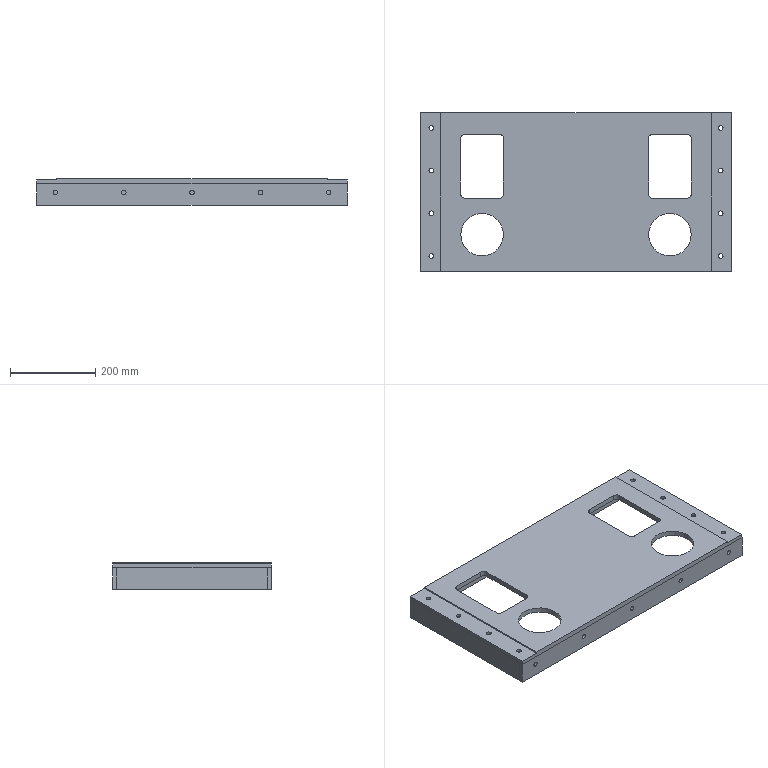Component | SolidWorks | MovingVerticalPlate2-1 | 6 solids | 125 faces | box 728 x 372 x 63 mm | volume 3861761 mm3 | cylinder 64 | plane 61 | commonest cylinder face diameters 18 x26 11 x26 20 x8 100 x4
build123d program:
from build123d import *

# Parameters (mm, degrees)
SKETCH1_W                                  = 728
SKETCH1_H                                  = 372
BOSS_EXTRUDE1_DEPTH                        = 12
SKETCH2_W                                  = 728
SKETCH2_H                                  = 10
BOSS_EXTRUDE2_DEPTH                        = 51
SKETCH3_W                                  = 10
SKETCH3_H                                  = 352
BOSS_EXTRUDE3_DEPTH                        = 51
SKETCH4_W                                  = 10
SKETCH4_H                                  = 352
BOSS_EXTRUDE4_DEPTH                        = 51
HOLE_SIZE_ACCORDING_TO_TYPE_1_OF_H_2_COUNT = 2
HOLE_SIZE_ACCORDING_TO_TYPE_1_OF_H_2_PITCH = 159.546
HOLE_SIZE_ACCORDING_TO_TYPE_1_OF_H_3_COUNT = 2
HOLE_SIZE_ACCORDING_TO_TYPE_1_OF_H_3_PITCH = 320
HOLE_SIZE_ACCORDING_TO_TYPE_1_OF_H_4_COUNT = 2
HOLE_SIZE_ACCORDING_TO_TYPE_1_OF_H_4_PITCH = 480
HOLE_SIZE_ACCORDING_TO_TYPE_1_OF_H_5_COUNT = 2
HOLE_SIZE_ACCORDING_TO_TYPE_1_OF_H_5_PITCH = 640
HOLE_SIZE_ACCORDING_TO_TYPE_2_OF_H_2_COUNT = 2
HOLE_SIZE_ACCORDING_TO_TYPE_2_OF_H_2_PITCH = 100
HOLE_SIZE_ACCORDING_TO_TYPE_2_OF_H_3_COUNT = 2
HOLE_SIZE_ACCORDING_TO_TYPE_2_OF_H_3_PITCH = 200
HOLE_SIZE_ACCORDING_TO_TYPE_2_OF_H_4_COUNT = 2
HOLE_SIZE_ACCORDING_TO_TYPE_2_OF_H_4_PITCH = 300
SKETCH9_R                                  = 50
SKETCH9_W                                  = 100
SKETCH9_H                                  = 150
CUT_EXTRUDE1_DEPTH                         = 412.938
FILLET1_R                                  = 10
SKETCH10_W                                 = 47
SKETCH10_H                                 = 3
CUT_EXTRUDE2_DEPTH                         = 525.26


with BuildPart() as part:
    # Sketch1 → Boss-Extrude1 (new body)
    with BuildSketch(Plane.XY):
        Rectangle(SKETCH1_W, SKETCH1_H)
    extrude(amount=BOSS_EXTRUDE1_DEPTH)

    # Sketch8 → Hole Size _According to_ Type 2 of Hexag (revolve, cut)
    with BuildSketch(Plane(origin=(-339, -150, 12), x_dir=(0, -1, 0), z_dir=(1, 0, 0))):
        Polygon((0, 0), (0, 12), (5.5, 12), (5.5, 3), (9, 3), (9, 0), align=None)
    hole_size_according_to_type_2_of_hexag = revolve(axis=Axis((-339, -150, 18.35), (0, 0, -1)), mode=Mode.SUBTRACT)

    # Hole Size _According to_ Type 2 of H 2: Hole Size _According to_ Type 2 of Hexag ×2
    with Locations(*[(0, i * HOLE_SIZE_ACCORDING_TO_TYPE_2_OF_H_2_PITCH, 0) for i in range(1, HOLE_SIZE_ACCORDING_TO_TYPE_2_OF_H_2_COUNT)]):
        add(hole_size_according_to_type_2_of_hexag, mode=Mode.SUBTRACT)

    # Hole Size _According to_ Type 2 of H 3: Hole Size _According to_ Type 2 of Hexag ×2
    with Locations(*[(0, i * HOLE_SIZE_ACCORDING_TO_TYPE_2_OF_H_3_PITCH, 0) for i in range(1, HOLE_SIZE_ACCORDING_TO_TYPE_2_OF_H_3_COUNT)]):
        add(hole_size_according_to_type_2_of_hexag, mode=Mode.SUBTRACT)

    # Hole Size _According to_ Type 2 of H 4: Hole Size _According to_ Type 2 of Hexag ×2
    with Locations(*[(0, i * HOLE_SIZE_ACCORDING_TO_TYPE_2_OF_H_4_PITCH, 0) for i in range(1, HOLE_SIZE_ACCORDING_TO_TYPE_2_OF_H_4_COUNT)]):
        add(hole_size_according_to_type_2_of_hexag, mode=Mode.SUBTRACT)

    # Mirror3: Hole Size _According to_ Type 2 of Hexag across plane
    add(hole_size_according_to_type_2_of_hexag.mirror(Plane(origin=(0, 0, 0), x_dir=(0, 0, 1), z_dir=(1, 0, 0))), mode=Mode.SUBTRACT)

    # Mirror3 copy 1 sketch → Mirror3 copy 1 (revolve, cut)
    with BuildSketch(Plane(origin=(339, -50, 12), x_dir=(0, -1, 0), z_dir=(-1, 0, 0))):
        Polygon((0, 0), (0, -12), (5.5, -12), (5.5, -3), (9, -3), (9, 0), align=None)
    revolve(axis=Axis((339, -50, 18.35), (0, 0, 1)), mode=Mode.SUBTRACT)

    # Mirror3 copy 2 sketch → Mirror3 copy 2 (revolve, cut)
    with BuildSketch(Plane(origin=(339, 50, 12), x_dir=(0, -1, 0), z_dir=(-1, 0, 0))):
        Polygon((0, 0), (0, -12), (5.5, -12), (5.5, -3), (9, -3), (9, 0), align=None)
    revolve(axis=Axis((339, 50, 18.35), (0, 0, 1)), mode=Mode.SUBTRACT)

    # Mirror3 copy 3 sketch → Mirror3 copy 3 (revolve, cut)
    with BuildSketch(Plane(origin=(339, 150, 12), x_dir=(0, -1, 0), z_dir=(-1, 0, 0))):
        Polygon((0, 0), (0, -12), (5.5, -12), (5.5, -3), (9, -3), (9, 0), align=None)
    revolve(axis=Axis((339, 150, 18.35), (0, 0, 1)), mode=Mode.SUBTRACT)

    # Sketch9 → Cut-Extrude1 (cut, through all)
    with BuildSketch(Plane.XY.offset(12)):
        with Locations((-220, -100)):
            Circle(SKETCH9_R)
        with Locations(Location((220, -100, 0), (0, 0, 180))):
            Circle(SKETCH9_R)
        with Locations((-220, 60)):
            Rectangle(SKETCH9_W, SKETCH9_H)
        with Locations((220, 60)):
            Rectangle(SKETCH9_W, SKETCH9_H)
    extrude(amount=-CUT_EXTRUDE1_DEPTH, mode=Mode.SUBTRACT)

    # Fillet1
    fillet1_edges = [part.edges().sort_by_distance(p)[0] for p in [
        (-270, -15, 6),
        (-270, 135, 6),
        (-170, 135, 6),
        (-170, -15, 6),
        (170, 135, 6),
        (270, 135, 6),
        (270, -15, 6),
        (170, -15, 6),
    ]]
    fillet(fillet1_edges, radius=FILLET1_R)

    # Sketch10 → Cut-Extrude2 (cut, through all)
    with BuildSketch(Plane(origin=(0, 186, 0), x_dir=(1, 0, 0), z_dir=(0, 1, 0))):
        with Locations((340.5, -1.5)):
            Rectangle(SKETCH10_W, SKETCH10_H)
        with Locations((-340.5, -1.5)):
            Rectangle(SKETCH10_W, SKETCH10_H)
    extrude(amount=-CUT_EXTRUDE2_DEPTH, mode=Mode.SUBTRACT)


with BuildPart() as body_2:
    # Sketch2 → Boss-Extrude2 (new body)
    with BuildSketch(Plane.XY.offset(12)):
        with Locations((0, 181)):
            Rectangle(SKETCH2_W, SKETCH2_H)
    extrude(amount=BOSS_EXTRUDE2_DEPTH)


with BuildPart() as body_3:
    # Sketch3 → Boss-Extrude3 (new body)
    with BuildSketch(Plane.XY.offset(12)):
        with Locations((-359, 0)):
            Rectangle(SKETCH3_W, SKETCH3_H)
    extrude(amount=BOSS_EXTRUDE3_DEPTH)


with BuildPart() as body_4:
    # Mirror1: mirrored copy
    add(body_2.part.mirror(Plane.ZX))

    # Sketch6 → Hole Size _According to_ Type 1 of Hexag (revolve, cut)
    with BuildSketch(Plane(origin=(-320, -176, 33), x_dir=(0, 0, 1), z_dir=(1, 0, 0))):
        Polygon((0, 0), (0, 10), (5.5, 10), (5.5, 3), (9, 3), (9, 0), align=None)
    hole_size_according_to_type_1_of_hexag = revolve(axis=Axis((-320, -169.65, 33), (0, -1, 0)), mode=Mode.SUBTRACT)

    # Hole Size _According to_ Type 1 of H 2: Hole Size _According to_ Type 1 of Hexag ×2
    with Locations(*[(i * HOLE_SIZE_ACCORDING_TO_TYPE_1_OF_H_2_PITCH, 0, 0) for i in range(1, HOLE_SIZE_ACCORDING_TO_TYPE_1_OF_H_2_COUNT)]):
        add(hole_size_according_to_type_1_of_hexag, mode=Mode.SUBTRACT)

    # Hole Size _According to_ Type 1 of H 3: Hole Size _According to_ Type 1 of Hexag ×2
    with Locations(*[(i * HOLE_SIZE_ACCORDING_TO_TYPE_1_OF_H_3_PITCH, 0, 0) for i in range(1, HOLE_SIZE_ACCORDING_TO_TYPE_1_OF_H_3_COUNT)]):
        add(hole_size_according_to_type_1_of_hexag, mode=Mode.SUBTRACT)

    # Hole Size _According to_ Type 1 of H 4: Hole Size _According to_ Type 1 of Hexag ×2
    with Locations(*[(i * HOLE_SIZE_ACCORDING_TO_TYPE_1_OF_H_4_PITCH, 0, 0) for i in range(1, HOLE_SIZE_ACCORDING_TO_TYPE_1_OF_H_4_COUNT)]):
        add(hole_size_according_to_type_1_of_hexag, mode=Mode.SUBTRACT)

    # Hole Size _According to_ Type 1 of H 5: Hole Size _According to_ Type 1 of Hexag ×2
    with Locations(*[(i * HOLE_SIZE_ACCORDING_TO_TYPE_1_OF_H_5_PITCH, 0, 0) for i in range(1, HOLE_SIZE_ACCORDING_TO_TYPE_1_OF_H_5_COUNT)]):
        add(hole_size_according_to_type_1_of_hexag, mode=Mode.SUBTRACT)


with BuildPart() as body_5:
    # Mirror2: mirrored copy
    add(body_3.part.mirror(Plane(origin=(0, 0, 0), x_dir=(0, 0, 1), z_dir=(1, 0, 0))))


with BuildPart() as body_6:
    # Sketch4 → Boss-Extrude4 (new body)
    with BuildSketch(Plane.XY.offset(63)):
        with Locations((99, 0)):
            Rectangle(SKETCH4_W, SKETCH4_H)
    extrude(amount=-BOSS_EXTRUDE4_DEPTH)


solid = Compound([part.part, body_2.part, body_3.part, body_4.part, body_5.part, body_6.part])

# Placed as in the assembly
solid = solid.moved(Location((-140, 234, -236), (-180, 0, 180)))